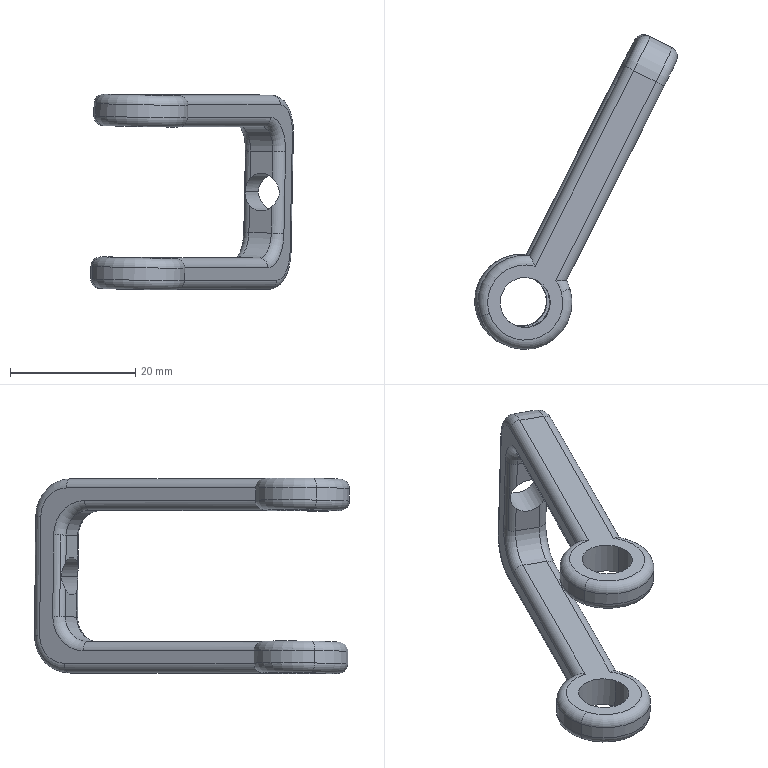Component | SolidWorks | ConnectingBlock-3 | 1 solid | 59 faces | volume 4352 mm3 | cylinder 29 | torus 20 | plane 10 | commonest cylinder face diameters 3 x13 8 x6 15 x6 6 x2 12 x2